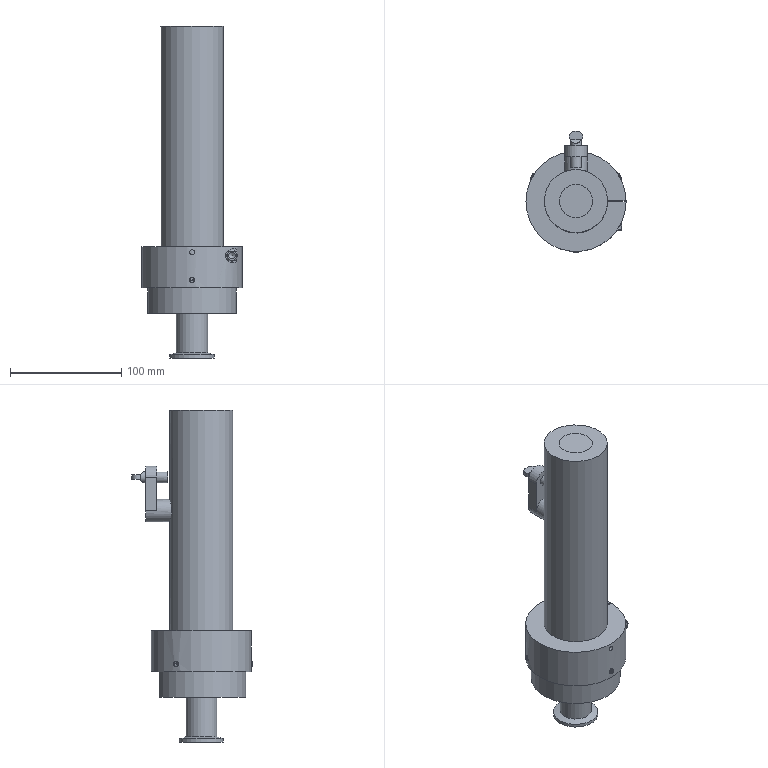Assembly | NX | mm | 17 component files | 18 solids | 286 faces | box 90 x 108.75 x 298.4 mm | volume 769287 mm3 | plane 178 | cylinder 74 | cone 26 | torus 7 | spline 1 | commonest cylinder face diameters 6 x14 10 x11 12 x7 7 x7 5 x6 80 x4 30 x3 20 x3
Bill of materials:
12 | 1 |  | Long solid cylinder with a small L-shaped side bracket near one end; the bracket ends in a short stepped pin or boss.
unnamed part 1 | 7 |  | Fastener shaped like a socket head cap screw: a cylindrical head with a hexagonal socket and a plain cylindrical shank with a chamfered tip.
CH3404.1-6 | 1 |  | Very thin flat ring (shim or thin washer shape) with a large central hole.
unnamed part 2 | 3 |  | Short solid cylindrical pin with chamfered ends and a shallow slot or notch cut across one end.
CH3404.1-1 | 1 |  | Thick round disc with a large central bore, six counterbored holes evenly spaced on a bolt circle, and a groove around the outer edge.
CH3404.1-2 | 1 |  | Flat ring shaped like a plain washer, thicker than the thin shim ring.
CH3404.1-3 | 1 |  | Plain solid disc: a short cylinder with flat faces and no features.
CH3404.1-5 | 1 |  | Split ring collar: a thick ring cut through by one radial slit, with a stepped bore, a counterbored clamping-style cross hole, and small radial holes.
CH3404.1-4 | 1 |  | Flanged hub: a large round flange with a flat on one edge and six holes, a central bore with a recessed ring, and a narrower cylindrical neck ending in a thin chamfered bottom flange.
Mates:
1. fix | CH3404_1-1 1 component
2. touch align | CH3404_1-2 1 face | CH3404_1-1 1 face
3. touch align | CH3404_1-2 1 datumplane | assembly datumplane
4. touch align | CH3404_1-2 1 face | assembly datumaxis
5. touch align | CH3404_1-3 1 face | CH3404_1-2 1 face
6. touch align | CH3404_1-3 1 | assembly datumplane
7. touch align | CH3404_1-3 1 face | assembly datumaxis
8. touch align | CH3404_1-4 1 face | CH3404_1-1 1 face
9. touch align | CH3404_1-4 1 | assembly datumplane
10. touch align | CH3404_1-4 1 face | CH3404_1-1 1 face
11. touch align | GB_T70_1_M6X25 7 face | CH3404_1-1 1 face
12. touch align | GB_T70_1_M6X25 7 face | CH3404_1-1 1 face
13. touch align | CH3404_1-6 1 face | CH3404_1-1 1 face
14. touch align | CH3404_1-6 1 face | assembly datumaxis
15. touch align | CH3404_1-5 1 face | CH3404_1-6 1 face
16. touch align | CH3404_1-5 1 face | assembly datumaxis
17. touch align | 12 1 face | CH3404_1-5 1 edge
18. touch align | 12 1 face | assembly datumaxis
19. touch align | 12 1 | assembly datumplane
20. touch align | GB_T70_1_M6X25 1 face | CH3404_1-5 1 face
21. touch align | GB-M5X8 3 face | CH3404_1-1 1 face
22. touch align | GB-M5X8 3 face | CH3404_1-5 1